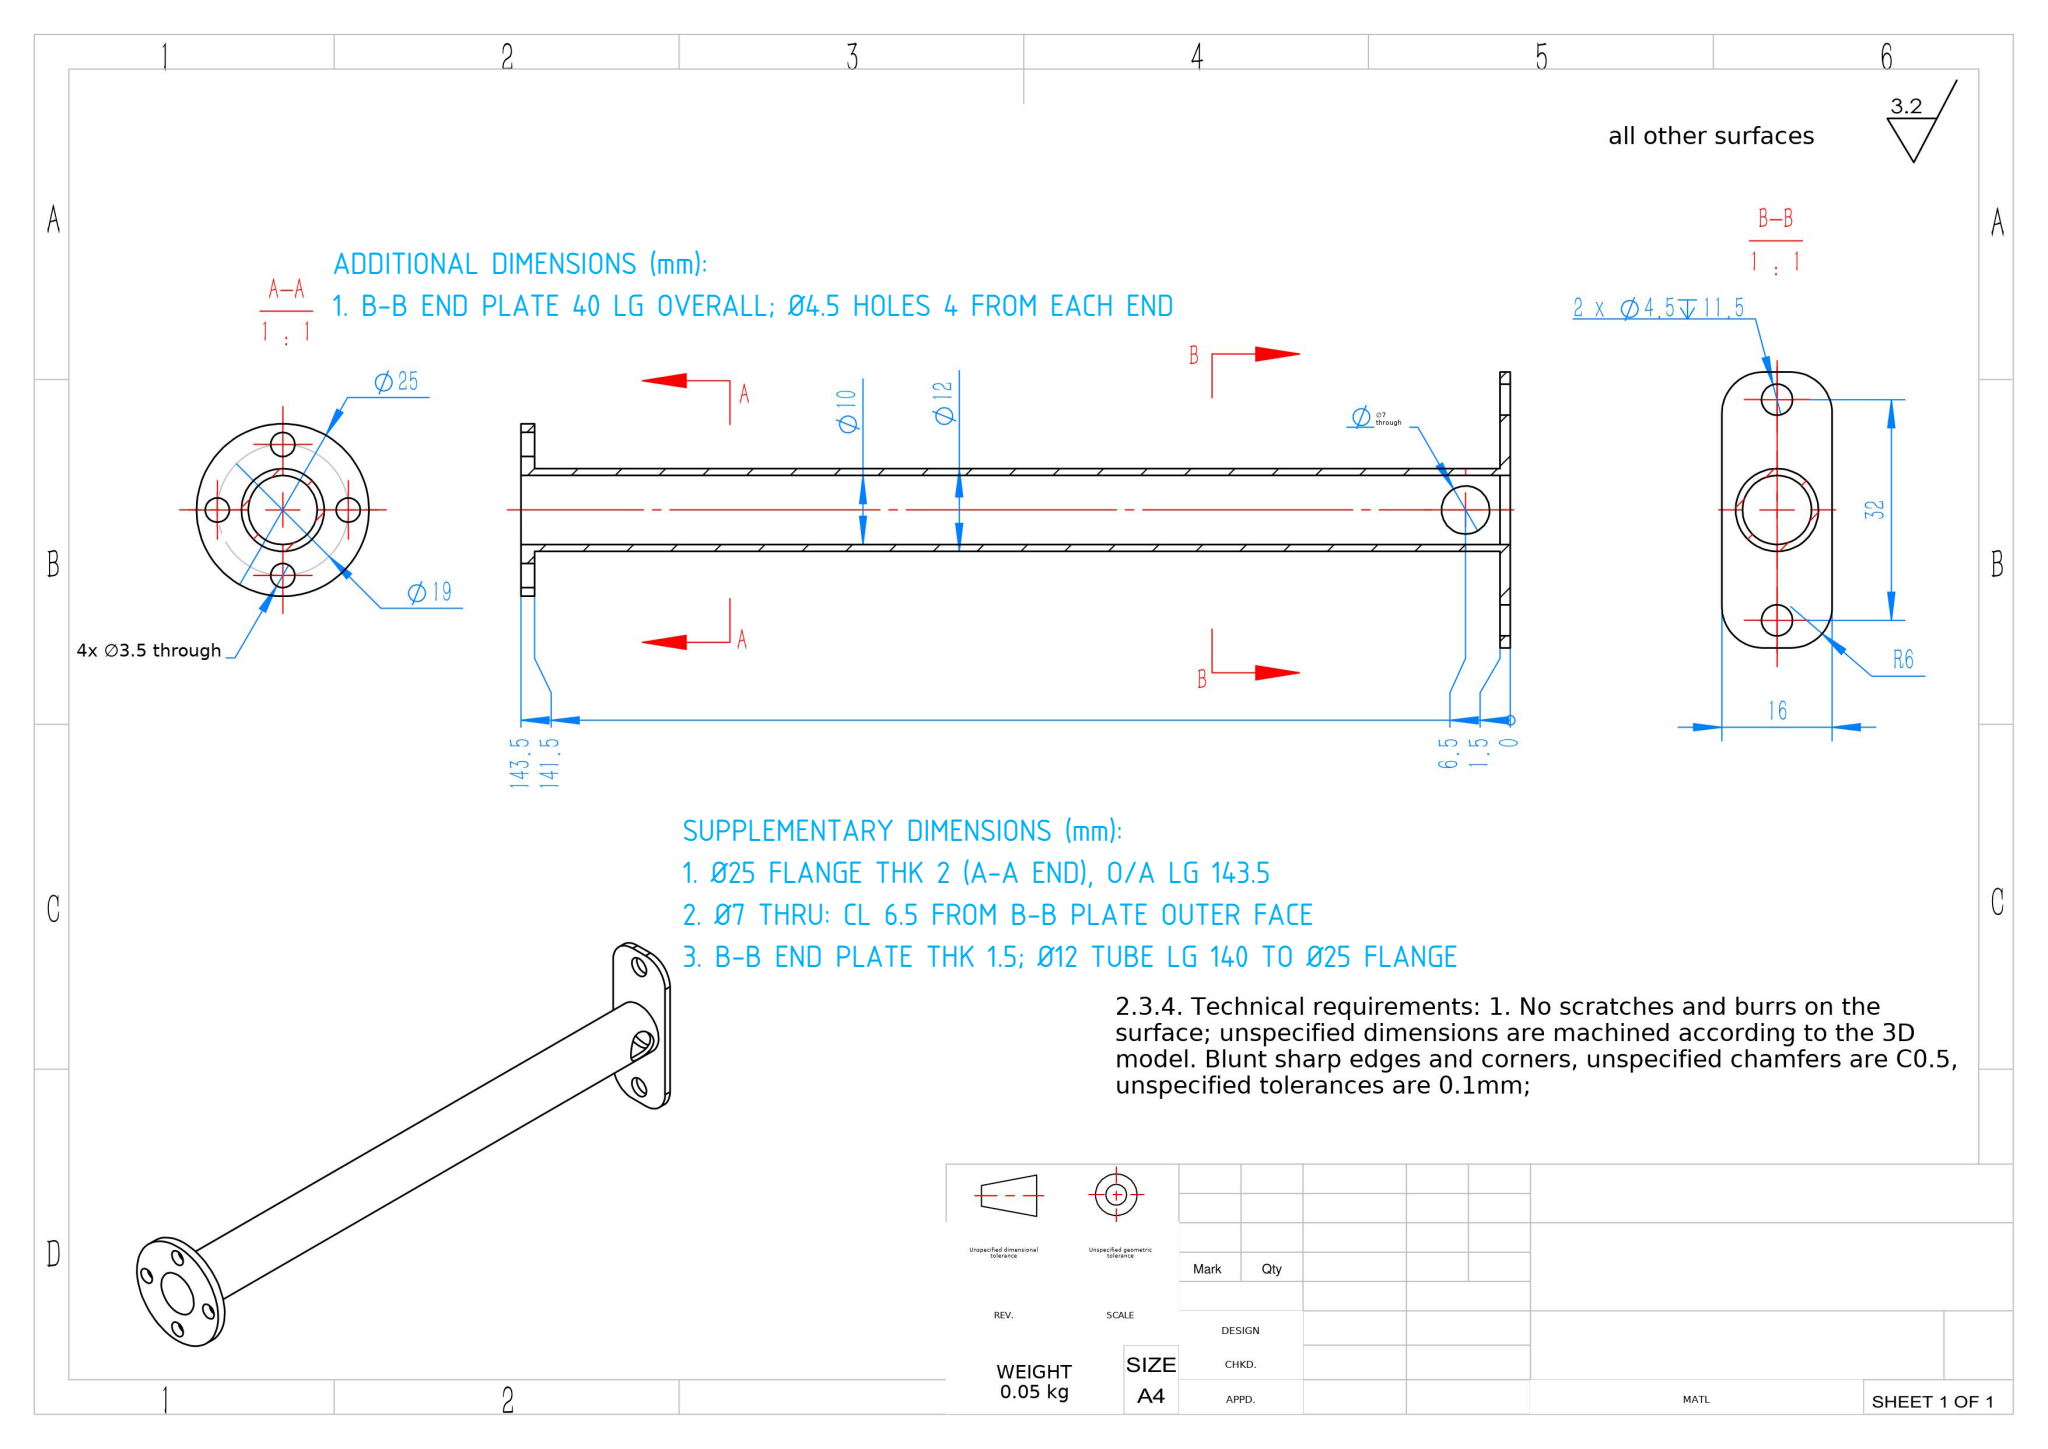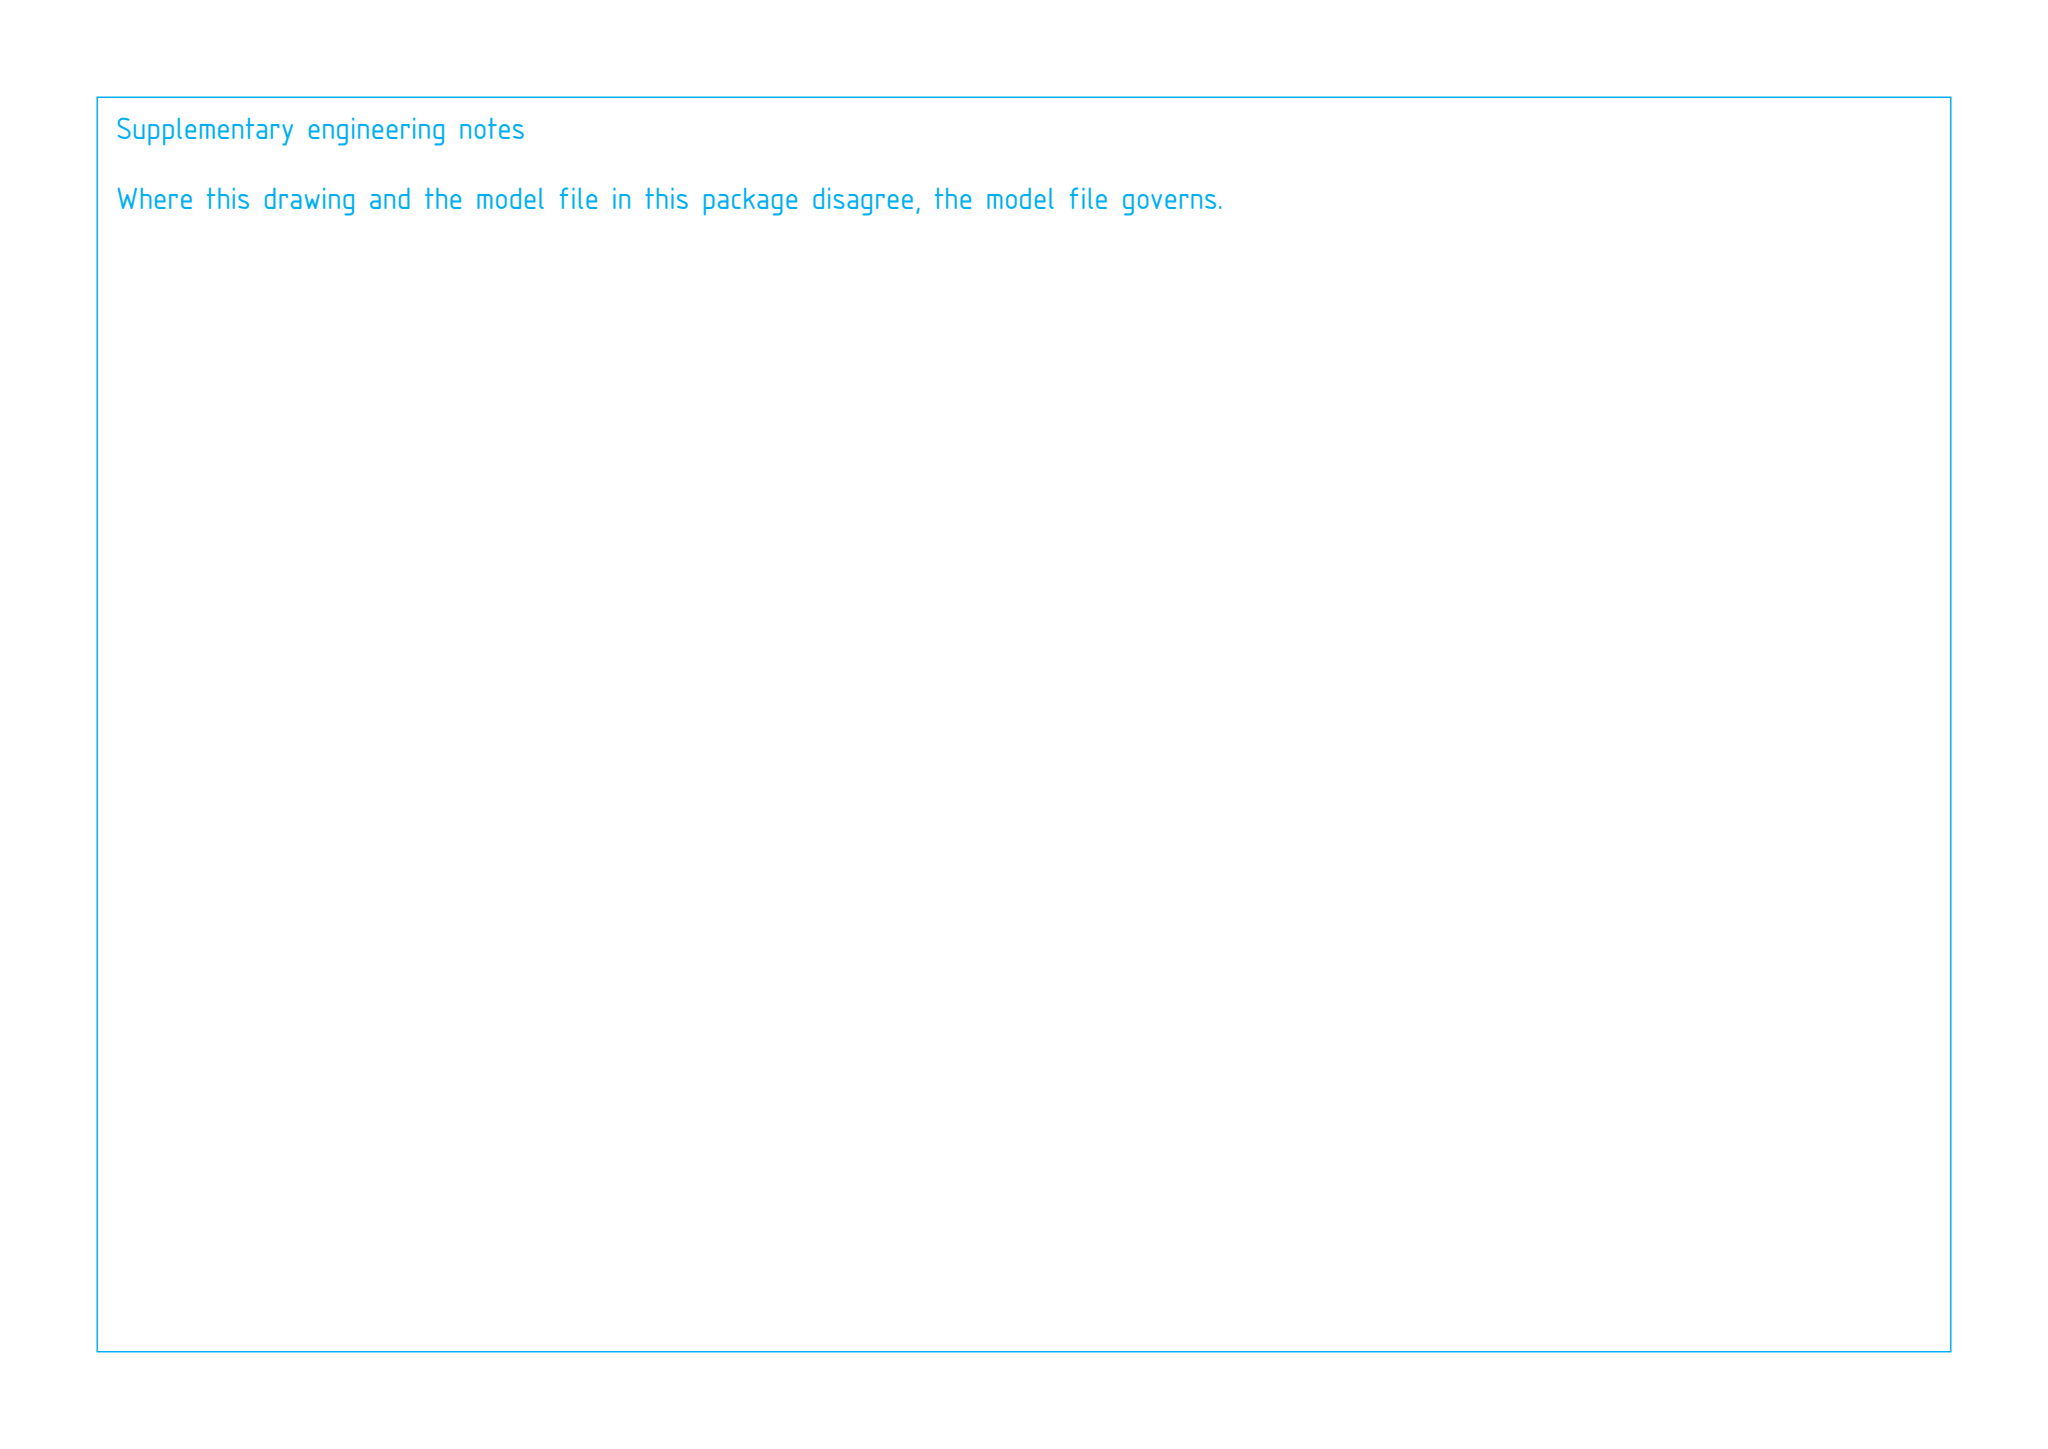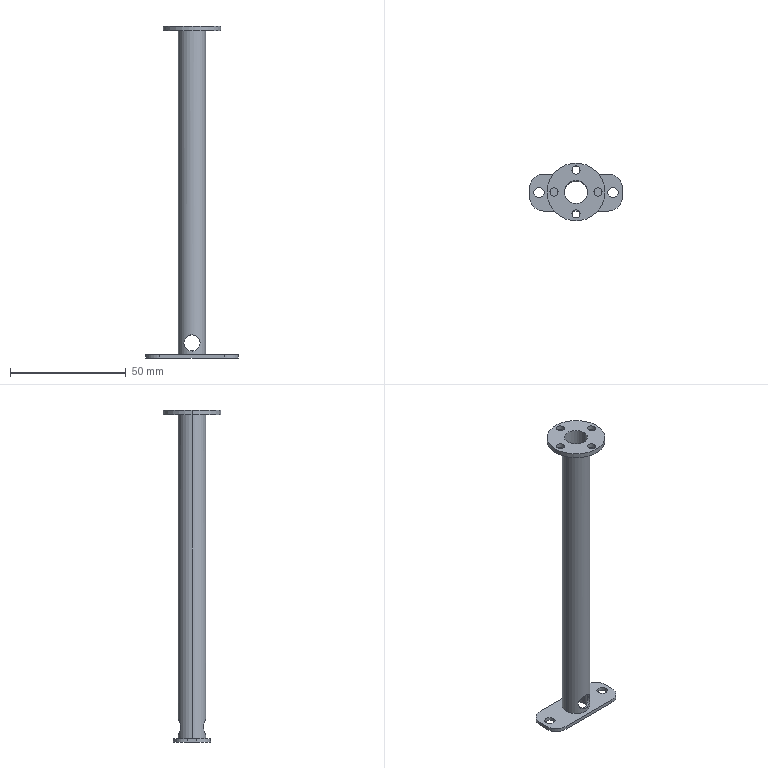Part | SolidWorks | mm | 1 solid | 36 faces | box 40 x 25 x 143.5 mm | volume 6252 mm3 | cylinder 28 | plane 8 | commonest cylinder face diameters 3.5 x8 12 x6 10 x4 7 x4 4.5 x4 25 x2